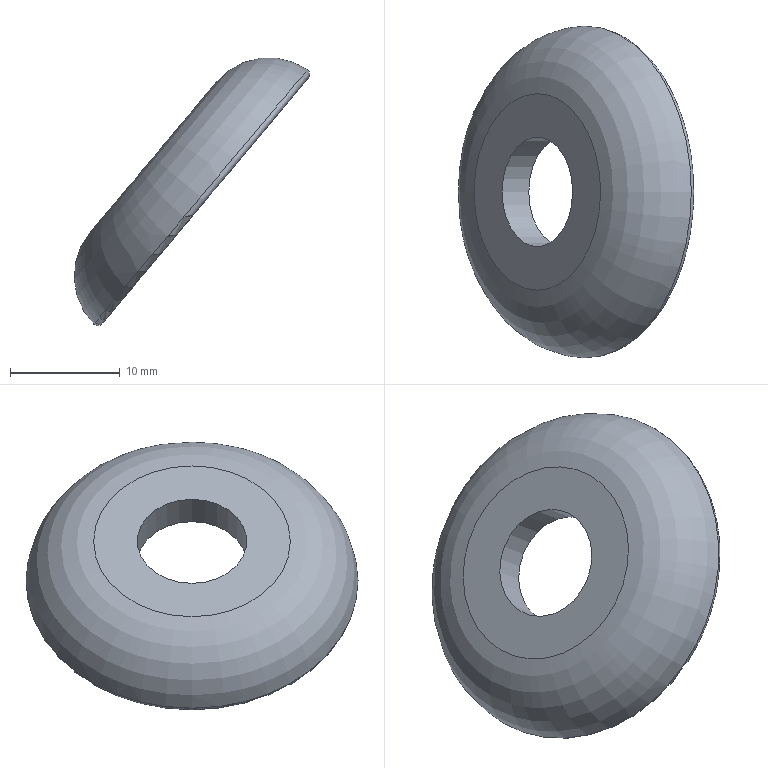Component | NX | BASEWASHER_2 | 1 solid | 9 faces | box 21.48 x 30.3 x 24.46 mm | volume 2198 mm3 | torus 4 | plane 3 | cylinder 2 | commonest cylinder face diameters 10 x1 24 x1
STEP:
#1=CARTESIAN_POINT('',(0.,0.,0.));
#2=DIRECTION('',(0.,0.,1.));
#3=DIRECTION('',(1.,0.,0.));
#4=AXIS2_PLACEMENT_3D('',#1,#2,#3);
#5=CARTESIAN_POINT('',(413.514,0.,-45.75));
#6=VERTEX_POINT('',#5);
#7=CARTESIAN_POINT('',(419.941,0.,-38.089));
#8=DIRECTION('',(0.766,0.,-0.6428));
#9=DIRECTION('',(-0.6428,0.,-0.766));
#10=AXIS2_PLACEMENT_3D('',#7,#8,#9);
#11=CIRCLE('',#10,10.);
#12=CARTESIAN_POINT('',(419.941,0.,-38.089));
#13=DIRECTION('',(0.766,0.,-0.6428));
#14=DIRECTION('',(-0.6428,0.,-0.766));
#15=AXIS2_PLACEMENT_3D('',#12,#13,#14);
#16=PLANE('',#15);
#17=CARTESIAN_POINT('',(-0.,0.));
#18=DIRECTION('',(1.,0.));
#19=AXIS2_PLACEMENT_2D('',#17,#18);
#20=CIRCLE('',#19,10.);
#21=(GEOMETRIC_REPRESENTATION_CONTEXT(2)PARAMETRIC_REPRESENTATION_CONTEXT()REPRESENTATION_CONTEXT('',''));
#22=DEFINITIONAL_REPRESENTATION('',(#20),#21);
#23=PCURVE('',#16,#22);
#24=CARTESIAN_POINT('',(421.473,0.,-39.375));
#25=DIRECTION('',(0.766,0.,-0.6428));
#26=DIRECTION('',(-0.6428,0.,-0.766));
#27=AXIS2_PLACEMENT_3D('',#24,#25,#26);
#28=TOROIDAL_SURFACE('',#27,10.,2.);
#29=CARTESIAN_POINT('',(0.,4.712));
#30=DIRECTION('',(1.,0.));
#31=VECTOR('',#30,1.);
#32=LINE('',#29,#31);
#33=(GEOMETRIC_REPRESENTATION_CONTEXT(2)PARAMETRIC_REPRESENTATION_CONTEXT()REPRESENTATION_CONTEXT('',''));
#34=DEFINITIONAL_REPRESENTATION('',(#32),#33);
#35=PCURVE('',#28,#34);
#36=SURFACE_CURVE('',#11,(#23,#35),.PCURVE_S1.);
#37=EDGE_CURVE('',#6,#6,#36,.T.);
#38=ORIENTED_EDGE('',*,*,#37,.T.);
#39=EDGE_LOOP('',(#38));
#40=FACE_BOUND('',#39,.T.);
#41=CARTESIAN_POINT('',(423.155,0.,-34.259));
#42=VERTEX_POINT('',#41);
#43=CARTESIAN_POINT('',(419.941,0.,-38.089));
#44=DIRECTION('',(-0.766,0.,0.6428));
#45=DIRECTION('',(0.6428,0.,0.766));
#46=AXIS2_PLACEMENT_3D('',#43,#44,#45);
#47=CIRCLE('',#46,5.);
#48=CARTESIAN_POINT('',(-5.,0.));
#49=CARTESIAN_POINT('',(-5.,8.66));
#50=CARTESIAN_POINT('',(2.5,4.33));
#51=CARTESIAN_POINT('',(10.,0.));
#52=CARTESIAN_POINT('',(2.5,-4.33));
#53=CARTESIAN_POINT('',(-5.,-8.66));
#54=CARTESIAN_POINT('',(-5.,0.));
#55=(BOUNDED_CURVE()B_SPLINE_CURVE(2,(#48,#49,#50,#51,#52,#53,#54),.UNSPECIFIED.,.T.,.F.)B_SPLINE_CURVE_WITH_KNOTS((1,2,2,2,2,1),(-2.094,0.,2.094,4.189,6.283,8.378),.UNSPECIFIED.)CURVE()GEOMETRIC_REPRESENTATION_ITEM()RATIONAL_B_SPLINE_CURVE((1.,0.5,1.,0.5,1.,0.5,1.))REPRESENTATION_ITEM(''));
#56=(GEOMETRIC_REPRESENTATION_CONTEXT(2)PARAMETRIC_REPRESENTATION_CONTEXT()REPRESENTATION_CONTEXT('',''));
#57=DEFINITIONAL_REPRESENTATION('',(#55),#56);
#58=PCURVE('',#16,#57);
#59=CARTESIAN_POINT('',(419.941,0.,-38.089));
#60=DIRECTION('',(-0.766,0.,0.6428));
#61=DIRECTION('',(0.6428,0.,0.766));
#62=AXIS2_PLACEMENT_3D('',#59,#60,#61);
#63=CYLINDRICAL_SURFACE('',#62,5.);
#64=CARTESIAN_POINT('',(0.,0.));
#65=DIRECTION('',(1.,0.));
#66=VECTOR('',#65,1.);
#67=LINE('',#64,#66);
#68=(GEOMETRIC_REPRESENTATION_CONTEXT(2)PARAMETRIC_REPRESENTATION_CONTEXT()REPRESENTATION_CONTEXT('',''));
#69=DEFINITIONAL_REPRESENTATION('',(#67),#68);
#70=PCURVE('',#63,#69);
#71=SURFACE_CURVE('',#47,(#58,#70),.PCURVE_S1.);
#72=EDGE_CURVE('',#42,#42,#71,.T.);
#73=ORIENTED_EDGE('',*,*,#72,.T.);
#74=EDGE_LOOP('',(#73));
#75=FACE_BOUND('',#74,.T.);
#76=ADVANCED_FACE('',(#40,#75),#16,.T.);
#77=CARTESIAN_POINT('',(423.278,0.,-29.173));
#78=VERTEX_POINT('',#77);
#79=CARTESIAN_POINT('',(411.74,0.,-42.924));
#80=VERTEX_POINT('',#79);
#81=CARTESIAN_POINT('',(417.509,0.,-36.049));
#82=DIRECTION('',(-0.766,0.,0.6428));
#83=DIRECTION('',(0.6428,0.,0.766));
#84=AXIS2_PLACEMENT_3D('',#81,#82,#83);
#85=CIRCLE('',#84,8.975);
#86=CARTESIAN_POINT('',(417.509,0.,-36.049));
#87=DIRECTION('',(-0.766,0.,0.6428));
#88=DIRECTION('',(0.6428,0.,0.766));
#89=AXIS2_PLACEMENT_3D('',#86,#87,#88);
#90=PLANE('',#89);
#91=CARTESIAN_POINT('',(0.,0.));
#92=DIRECTION('',(1.,0.));
#93=AXIS2_PLACEMENT_2D('',#91,#92);
#94=CIRCLE('',#93,8.975);
#95=(GEOMETRIC_REPRESENTATION_CONTEXT(2)PARAMETRIC_REPRESENTATION_CONTEXT()REPRESENTATION_CONTEXT('',''));
#96=DEFINITIONAL_REPRESENTATION('',(#94),#95);
#97=PCURVE('',#90,#96);
#98=CARTESIAN_POINT('',(422.259,0.,-40.034));
#99=DIRECTION('',(0.766,0.,-0.6428));
#100=DIRECTION('',(-0.6428,0.,-0.766));
#101=AXIS2_PLACEMENT_3D('',#98,#99,#100);
#102=TOROIDAL_SURFACE('',#101,8.975,6.2);
#103=CARTESIAN_POINT('',(3.142,4.712));
#104=DIRECTION('',(-1.,0.));
#105=VECTOR('',#104,1.);
#106=LINE('',#103,#105);
#107=(GEOMETRIC_REPRESENTATION_CONTEXT(2)PARAMETRIC_REPRESENTATION_CONTEXT()REPRESENTATION_CONTEXT('',''));
#108=DEFINITIONAL_REPRESENTATION('',(#106),#107);
#109=PCURVE('',#102,#108);
#110=SURFACE_CURVE('',#85,(#97,#109),.PCURVE_S1.);
#111=EDGE_CURVE('',#78,#80,#110,.T.);
#112=ORIENTED_EDGE('',*,*,#111,.T.);
#113=CARTESIAN_POINT('',(417.509,0.,-36.049));
#114=DIRECTION('',(-0.766,0.,0.6428));
#115=DIRECTION('',(0.6428,0.,0.766));
#116=AXIS2_PLACEMENT_3D('',#113,#114,#115);
#117=CIRCLE('',#116,8.975);
#118=CARTESIAN_POINT('',(0.,0.));
#119=DIRECTION('',(1.,0.));
#120=AXIS2_PLACEMENT_2D('',#118,#119);
#121=CIRCLE('',#120,8.975);
#122=(GEOMETRIC_REPRESENTATION_CONTEXT(2)PARAMETRIC_REPRESENTATION_CONTEXT()REPRESENTATION_CONTEXT('',''));
#123=DEFINITIONAL_REPRESENTATION('',(#121),#122);
#124=PCURVE('',#90,#123);
#125=CARTESIAN_POINT('',(9.425,4.712));
#126=DIRECTION('',(-1.,0.));
#127=VECTOR('',#126,1.);
#128=LINE('',#125,#127);
#129=(GEOMETRIC_REPRESENTATION_CONTEXT(2)PARAMETRIC_REPRESENTATION_CONTEXT()REPRESENTATION_CONTEXT('',''));
#130=DEFINITIONAL_REPRESENTATION('',(#128),#129);
#131=PCURVE('',#102,#130);
#132=SURFACE_CURVE('',#117,(#124,#131),.PCURVE_S1.);
#133=EDGE_CURVE('',#80,#78,#132,.T.);
#134=ORIENTED_EDGE('',*,*,#133,.T.);
#135=EDGE_LOOP('',(#112,#134));
#136=FACE_BOUND('',#135,.T.);
#137=CARTESIAN_POINT('',(420.723,0.,-32.218));
#138=VERTEX_POINT('',#137);
#139=CARTESIAN_POINT('',(417.509,0.,-36.049));
#140=DIRECTION('',(0.766,0.,-0.6428));
#141=DIRECTION('',(0.6428,0.,0.766));
#142=AXIS2_PLACEMENT_3D('',#139,#140,#141);
#143=CIRCLE('',#142,5.);
#144=CARTESIAN_POINT('',(5.,0.));
#145=CARTESIAN_POINT('',(5.,-8.66));
#146=CARTESIAN_POINT('',(-2.5,-4.33));
#147=CARTESIAN_POINT('',(-10.,-0.));
#148=CARTESIAN_POINT('',(-2.5,4.33));
#149=CARTESIAN_POINT('',(5.,8.66));
#150=CARTESIAN_POINT('',(5.,0.));
#151=(BOUNDED_CURVE()B_SPLINE_CURVE(2,(#144,#145,#146,#147,#148,#149,#150),.UNSPECIFIED.,.T.,.F.)B_SPLINE_CURVE_WITH_KNOTS((1,2,2,2,2,1),(-2.094,0.,2.094,4.189,6.283,8.378),.UNSPECIFIED.)CURVE()GEOMETRIC_REPRESENTATION_ITEM()RATIONAL_B_SPLINE_CURVE((1.,0.5,1.,0.5,1.,0.5,1.))REPRESENTATION_ITEM(''));
#152=(GEOMETRIC_REPRESENTATION_CONTEXT(2)PARAMETRIC_REPRESENTATION_CONTEXT()REPRESENTATION_CONTEXT('',''));
#153=DEFINITIONAL_REPRESENTATION('',(#151),#152);
#154=PCURVE('',#90,#153);
#155=CARTESIAN_POINT('',(6.283,3.175));
#156=DIRECTION('',(-1.,0.));
#157=VECTOR('',#156,1.);
#158=LINE('',#155,#157);
#159=(GEOMETRIC_REPRESENTATION_CONTEXT(2)PARAMETRIC_REPRESENTATION_CONTEXT()REPRESENTATION_CONTEXT('',''));
#160=DEFINITIONAL_REPRESENTATION('',(#158),#159);
#161=PCURVE('',#63,#160);
#162=SURFACE_CURVE('',#143,(#154,#161),.PCURVE_S1.);
#163=EDGE_CURVE('',#138,#138,#162,.T.);
#164=ORIENTED_EDGE('',*,*,#163,.T.);
#165=EDGE_LOOP('',(#164));
#166=FACE_BOUND('',#165,.T.);
#167=ADVANCED_FACE('',(#136,#166),#90,.T.);
#168=ORIENTED_EDGE('',*,*,#163,.T.);
#169=CARTESIAN_POINT('',(423.155,-0.,-34.259));
#170=CARTESIAN_POINT('',(420.723,-0.,-32.218));
#171=B_SPLINE_CURVE_WITH_KNOTS('',1,(#169,#170),.UNSPECIFIED.,.F.,.F.,(2,2),(0.,3.175),.PIECEWISE_BEZIER_KNOTS.);
#172=CARTESIAN_POINT('',(0.,0.));
#173=DIRECTION('',(0.,1.));
#174=VECTOR('',#173,1.);
#175=LINE('',#172,#174);
#176=(GEOMETRIC_REPRESENTATION_CONTEXT(2)PARAMETRIC_REPRESENTATION_CONTEXT()REPRESENTATION_CONTEXT('',''));
#177=DEFINITIONAL_REPRESENTATION('',(#175),#176);
#178=PCURVE('',#63,#177);
#179=CARTESIAN_POINT('',(6.283,0.));
#180=DIRECTION('',(0.,1.));
#181=VECTOR('',#180,1.);
#182=LINE('',#179,#181);
#183=(GEOMETRIC_REPRESENTATION_CONTEXT(2)PARAMETRIC_REPRESENTATION_CONTEXT()REPRESENTATION_CONTEXT('',''));
#184=DEFINITIONAL_REPRESENTATION('',(#182),#183);
#185=PCURVE('',#63,#184);
#186=SEAM_CURVE('',#171,(#178,#185),.PCURVE_S1.);
#187=EDGE_CURVE('',#42,#138,#186,.T.);
#188=ORIENTED_EDGE('',*,*,#187,.F.);
#189=ORIENTED_EDGE('',*,*,#72,.T.);
#190=ORIENTED_EDGE('',*,*,#187,.T.);
#191=EDGE_LOOP('',(#168,#188,#189,#190));
#192=FACE_BOUND('',#191,.F.);
#193=ADVANCED_FACE('',(#192),#63,.F.);
#194=CARTESIAN_POINT('',(414.143,0.,-48.889));
#195=VERTEX_POINT('',#194);
#196=CARTESIAN_POINT('',(421.857,0.,-39.696));
#197=DIRECTION('',(0.766,0.,-0.6428));
#198=DIRECTION('',(-0.6428,0.,-0.766));
#199=AXIS2_PLACEMENT_3D('',#196,#197,#198);
#200=CIRCLE('',#199,12.);
#201=CARTESIAN_POINT('',(419.941,0.,-38.089));
#202=DIRECTION('',(0.766,0.,-0.6428));
#203=DIRECTION('',(-0.6428,0.,-0.766));
#204=AXIS2_PLACEMENT_3D('',#201,#202,#203);
#205=CYLINDRICAL_SURFACE('',#204,12.);
#206=CARTESIAN_POINT('',(0.,2.5));
#207=DIRECTION('',(1.,0.));
#208=VECTOR('',#207,1.);
#209=LINE('',#206,#208);
#210=(GEOMETRIC_REPRESENTATION_CONTEXT(2)PARAMETRIC_REPRESENTATION_CONTEXT()REPRESENTATION_CONTEXT('',''));
#211=DEFINITIONAL_REPRESENTATION('',(#209),#210);
#212=PCURVE('',#205,#211);
#213=CARTESIAN_POINT('',(421.857,0.,-39.696));
#214=DIRECTION('',(0.766,0.,-0.6428));
#215=DIRECTION('',(-0.6428,0.,-0.766));
#216=AXIS2_PLACEMENT_3D('',#213,#214,#215);
#217=TOROIDAL_SURFACE('',#216,12.5,0.5);
#218=CARTESIAN_POINT('',(0.,9.425));
#219=DIRECTION('',(1.,0.));
#220=VECTOR('',#219,1.);
#221=LINE('',#218,#220);
#222=(GEOMETRIC_REPRESENTATION_CONTEXT(2)PARAMETRIC_REPRESENTATION_CONTEXT()REPRESENTATION_CONTEXT('',''));
#223=DEFINITIONAL_REPRESENTATION('',(#221),#222);
#224=PCURVE('',#217,#223);
#225=SURFACE_CURVE('',#200,(#212,#224),.PCURVE_S1.);
#226=EDGE_CURVE('',#195,#195,#225,.T.);
#227=ORIENTED_EDGE('',*,*,#226,.F.);
#228=CARTESIAN_POINT('',(413.76,0.,-48.568));
#229=VERTEX_POINT('',#228);
#230=CARTESIAN_POINT('',(413.76,-0.,-48.568));
#231=CARTESIAN_POINT('',(414.143,-0.,-48.889));
#232=B_SPLINE_CURVE_WITH_KNOTS('',1,(#230,#231),.UNSPECIFIED.,.F.,.F.,(2,2),(2.,2.5),.PIECEWISE_BEZIER_KNOTS.);
#233=CARTESIAN_POINT('',(0.,0.));
#234=DIRECTION('',(0.,1.));
#235=VECTOR('',#234,1.);
#236=LINE('',#233,#235);
#237=(GEOMETRIC_REPRESENTATION_CONTEXT(2)PARAMETRIC_REPRESENTATION_CONTEXT()REPRESENTATION_CONTEXT('',''));
#238=DEFINITIONAL_REPRESENTATION('',(#236),#237);
#239=PCURVE('',#205,#238);
#240=CARTESIAN_POINT('',(6.283,0.));
#241=DIRECTION('',(0.,1.));
#242=VECTOR('',#241,1.);
#243=LINE('',#240,#242);
#244=(GEOMETRIC_REPRESENTATION_CONTEXT(2)PARAMETRIC_REPRESENTATION_CONTEXT()REPRESENTATION_CONTEXT('',''));
#245=DEFINITIONAL_REPRESENTATION('',(#243),#244);
#246=PCURVE('',#205,#245);
#247=SEAM_CURVE('',#232,(#239,#246),.PCURVE_S1.);
#248=EDGE_CURVE('',#229,#195,#247,.T.);
#249=ORIENTED_EDGE('',*,*,#248,.F.);
#250=CARTESIAN_POINT('',(421.473,0.,-39.375));
#251=DIRECTION('',(-0.766,0.,0.6428));
#252=DIRECTION('',(-0.6428,0.,-0.766));
#253=AXIS2_PLACEMENT_3D('',#250,#251,#252);
#254=CIRCLE('',#253,12.);
#255=CARTESIAN_POINT('',(6.283,2.));
#256=DIRECTION('',(-1.,0.));
#257=VECTOR('',#256,1.);
#258=LINE('',#255,#257);
#259=(GEOMETRIC_REPRESENTATION_CONTEXT(2)PARAMETRIC_REPRESENTATION_CONTEXT()REPRESENTATION_CONTEXT('',''));
#260=DEFINITIONAL_REPRESENTATION('',(#258),#259);
#261=PCURVE('',#205,#260);
#262=CARTESIAN_POINT('',(6.283,6.283));
#263=DIRECTION('',(-1.,0.));
#264=VECTOR('',#263,1.);
#265=LINE('',#262,#264);
#266=(GEOMETRIC_REPRESENTATION_CONTEXT(2)PARAMETRIC_REPRESENTATION_CONTEXT()REPRESENTATION_CONTEXT('',''));
#267=DEFINITIONAL_REPRESENTATION('',(#265),#266);
#268=PCURVE('',#28,#267);
#269=SURFACE_CURVE('',#254,(#261,#268),.PCURVE_S1.);
#270=EDGE_CURVE('',#229,#229,#269,.T.);
#271=ORIENTED_EDGE('',*,*,#270,.F.);
#272=ORIENTED_EDGE('',*,*,#248,.T.);
#273=EDGE_LOOP('',(#227,#249,#271,#272));
#274=FACE_BOUND('',#273,.F.);
#275=ADVANCED_FACE('',(#274),#205,.F.);
#276=CARTESIAN_POINT('',(414.205,0.,-49.593));
#277=VERTEX_POINT('',#276);
#278=CARTESIAN_POINT('',(422.24,0.,-40.018));
#279=DIRECTION('',(-0.766,0.,0.6428));
#280=DIRECTION('',(-0.6428,0.,-0.766));
#281=AXIS2_PLACEMENT_3D('',#278,#279,#280);
#282=CIRCLE('',#281,12.5);
#283=CARTESIAN_POINT('',(414.526,0.,-49.21));
#284=DIRECTION('',(0.766,0.,-0.6428));
#285=DIRECTION('',(-0.6428,0.,-0.766));
#286=AXIS2_PLACEMENT_3D('',#283,#284,#285);
#287=PLANE('',#286);
#288=CARTESIAN_POINT('',(0.5,0.));
#289=CARTESIAN_POINT('',(0.5,-21.651));
#290=CARTESIAN_POINT('',(-18.25,-10.825));
#291=CARTESIAN_POINT('',(-37.,-0.));
#292=CARTESIAN_POINT('',(-18.25,10.825));
#293=CARTESIAN_POINT('',(0.5,21.651));
#294=CARTESIAN_POINT('',(0.5,0.));
#295=(BOUNDED_CURVE()B_SPLINE_CURVE(2,(#288,#289,#290,#291,#292,#293,#294),.UNSPECIFIED.,.T.,.F.)B_SPLINE_CURVE_WITH_KNOTS((1,2,2,2,2,1),(-2.094,0.,2.094,4.189,6.283,8.378),.UNSPECIFIED.)CURVE()GEOMETRIC_REPRESENTATION_ITEM()RATIONAL_B_SPLINE_CURVE((1.,0.5,1.,0.5,1.,0.5,1.))REPRESENTATION_ITEM(''));
#296=(GEOMETRIC_REPRESENTATION_CONTEXT(2)PARAMETRIC_REPRESENTATION_CONTEXT()REPRESENTATION_CONTEXT('',''));
#297=DEFINITIONAL_REPRESENTATION('',(#295),#296);
#298=PCURVE('',#287,#297);
#299=CARTESIAN_POINT('',(6.283,7.854));
#300=DIRECTION('',(-1.,0.));
#301=VECTOR('',#300,1.);
#302=LINE('',#299,#301);
#303=(GEOMETRIC_REPRESENTATION_CONTEXT(2)PARAMETRIC_REPRESENTATION_CONTEXT()REPRESENTATION_CONTEXT('',''));
#304=DEFINITIONAL_REPRESENTATION('',(#302),#303);
#305=PCURVE('',#217,#304);
#306=SURFACE_CURVE('',#282,(#298,#305),.PCURVE_S1.);
#307=EDGE_CURVE('',#277,#277,#306,.T.);
#308=ORIENTED_EDGE('',*,*,#307,.T.);
#309=EDGE_LOOP('',(#308));
#310=FACE_BOUND('',#309,.T.);
#311=CARTESIAN_POINT('',(412.822,0.,-51.241));
#312=VERTEX_POINT('',#311);
#313=CARTESIAN_POINT('',(422.24,0.,-40.018));
#314=DIRECTION('',(0.766,0.,-0.6428));
#315=DIRECTION('',(-0.6428,0.,-0.766));
#316=AXIS2_PLACEMENT_3D('',#313,#314,#315);
#317=CIRCLE('',#316,14.651);
#318=CARTESIAN_POINT('',(-12.,0.));
#319=DIRECTION('',(1.,0.));
#320=AXIS2_PLACEMENT_2D('',#318,#319);
#321=CIRCLE('',#320,14.651);
#322=(GEOMETRIC_REPRESENTATION_CONTEXT(2)PARAMETRIC_REPRESENTATION_CONTEXT()REPRESENTATION_CONTEXT('',''));
#323=DEFINITIONAL_REPRESENTATION('',(#321),#322);
#324=PCURVE('',#287,#323);
#325=CARTESIAN_POINT('',(421.857,0.,-39.696));
#326=DIRECTION('',(0.766,0.,-0.6428));
#327=DIRECTION('',(-0.6428,0.,-0.766));
#328=AXIS2_PLACEMENT_3D('',#325,#326,#327);
#329=TOROIDAL_SURFACE('',#328,14.651,0.5);
#330=CARTESIAN_POINT('',(0.,7.854));
#331=DIRECTION('',(1.,0.));
#332=VECTOR('',#331,1.);
#333=LINE('',#330,#332);
#334=(GEOMETRIC_REPRESENTATION_CONTEXT(2)PARAMETRIC_REPRESENTATION_CONTEXT()REPRESENTATION_CONTEXT('',''));
#335=DEFINITIONAL_REPRESENTATION('',(#333),#334);
#336=PCURVE('',#329,#335);
#337=SURFACE_CURVE('',#317,(#324,#336),.PCURVE_S1.);
#338=EDGE_CURVE('',#312,#312,#337,.T.);
#339=ORIENTED_EDGE('',*,*,#338,.T.);
#340=EDGE_LOOP('',(#339));
#341=FACE_BOUND('',#340,.T.);
#342=ADVANCED_FACE('',(#310,#341),#287,.T.);
#343=ORIENTED_EDGE('',*,*,#37,.T.);
#344=CARTESIAN_POINT('',(413.514,0.,-45.75));
#345=CARTESIAN_POINT('',(413.17,0.,-46.159));
#346=CARTESIAN_POINT('',(412.965,0.,-46.668));
#347=CARTESIAN_POINT('',(412.927,0.,-47.221));
#348=CARTESIAN_POINT('',(413.061,0.,-47.759));
#349=CARTESIAN_POINT('',(413.35,0.,-48.224));
#350=CARTESIAN_POINT('',(413.76,0.,-48.568));
#351=(BOUNDED_CURVE()B_SPLINE_CURVE(6,(#344,#345,#346,#347,#348,#349,#350),.UNSPECIFIED.,.F.,.F.)B_SPLINE_CURVE_WITH_KNOTS((7,7),(4.712,6.283),.PIECEWISE_BEZIER_KNOTS.)CURVE()GEOMETRIC_REPRESENTATION_ITEM()RATIONAL_B_SPLINE_CURVE((1.031,1.01,0.9979,0.994,0.9979,1.01,1.031))REPRESENTATION_ITEM(''));
#352=CARTESIAN_POINT('',(6.283,0.));
#353=DIRECTION('',(0.,1.));
#354=VECTOR('',#353,1.);
#355=LINE('',#352,#354);
#356=(GEOMETRIC_REPRESENTATION_CONTEXT(2)PARAMETRIC_REPRESENTATION_CONTEXT()REPRESENTATION_CONTEXT('',''));
#357=DEFINITIONAL_REPRESENTATION('',(#355),#356);
#358=PCURVE('',#28,#357);
#359=CARTESIAN_POINT('',(0.,0.));
#360=DIRECTION('',(0.,1.));
#361=VECTOR('',#360,1.);
#362=LINE('',#359,#361);
#363=(GEOMETRIC_REPRESENTATION_CONTEXT(2)PARAMETRIC_REPRESENTATION_CONTEXT()REPRESENTATION_CONTEXT('',''));
#364=DEFINITIONAL_REPRESENTATION('',(#362),#363);
#365=PCURVE('',#28,#364);
#366=SEAM_CURVE('',#351,(#358,#365),.PCURVE_S1.);
#367=EDGE_CURVE('',#6,#229,#366,.T.);
#368=ORIENTED_EDGE('',*,*,#367,.T.);
#369=ORIENTED_EDGE('',*,*,#270,.T.);
#370=ORIENTED_EDGE('',*,*,#367,.F.);
#371=EDGE_LOOP('',(#343,#368,#369,#370));
#372=FACE_BOUND('',#371,.F.);
#373=ADVANCED_FACE('',(#372),#28,.F.);
#374=CARTESIAN_POINT('',(412.084,0.,-51.271));
#375=VERTEX_POINT('',#374);
#376=CARTESIAN_POINT('',(421.821,0.,-39.667));
#377=DIRECTION('',(-0.766,0.,0.6428));
#378=DIRECTION('',(-0.6428,0.,-0.766));
#379=AXIS2_PLACEMENT_3D('',#376,#377,#378);
#380=CIRCLE('',#379,15.149);
#381=CARTESIAN_POINT('',(6.283,6.191));
#382=DIRECTION('',(-1.,0.));
#383=VECTOR('',#382,1.);
#384=LINE('',#381,#383);
#385=(GEOMETRIC_REPRESENTATION_CONTEXT(2)PARAMETRIC_REPRESENTATION_CONTEXT()REPRESENTATION_CONTEXT('',''));
#386=DEFINITIONAL_REPRESENTATION('',(#384),#385);
#387=PCURVE('',#102,#386);
#388=CARTESIAN_POINT('',(6.283,6.191));
#389=DIRECTION('',(-1.,0.));
#390=VECTOR('',#389,1.);
#391=LINE('',#388,#390);
#392=(GEOMETRIC_REPRESENTATION_CONTEXT(2)PARAMETRIC_REPRESENTATION_CONTEXT()REPRESENTATION_CONTEXT('',''));
#393=DEFINITIONAL_REPRESENTATION('',(#391),#392);
#394=PCURVE('',#329,#393);
#395=SURFACE_CURVE('',#380,(#387,#394),.PCURVE_S1.);
#396=EDGE_CURVE('',#375,#375,#395,.T.);
#397=ORIENTED_EDGE('',*,*,#396,.T.);
#398=CARTESIAN_POINT('',(411.74,-0.,-42.924));
#399=CARTESIAN_POINT('',(410.74,-0.,-44.116));
#400=CARTESIAN_POINT('',(410.119,-0.,-45.58));
#401=CARTESIAN_POINT('',(409.948,-0.,-47.179));
#402=CARTESIAN_POINT('',(410.249,-0.,-48.757));
#403=CARTESIAN_POINT('',(410.989,-0.,-50.165));
#404=CARTESIAN_POINT('',(412.084,-0.,-51.271));
#405=(BOUNDED_CURVE()B_SPLINE_CURVE(6,(#398,#399,#400,#401,#402,#403,#404),.UNSPECIFIED.,.F.,.F.)B_SPLINE_CURVE_WITH_KNOTS((7,7),(4.712,6.191),.PIECEWISE_BEZIER_KNOTS.)CURVE()GEOMETRIC_REPRESENTATION_ITEM()RATIONAL_B_SPLINE_CURVE((1.028,1.009,0.9982,0.9946,0.9982,1.009,1.028))REPRESENTATION_ITEM(''));
#406=CARTESIAN_POINT('',(0.,0.));
#407=DIRECTION('',(0.,1.));
#408=VECTOR('',#407,1.);
#409=LINE('',#406,#408);
#410=(GEOMETRIC_REPRESENTATION_CONTEXT(2)PARAMETRIC_REPRESENTATION_CONTEXT()REPRESENTATION_CONTEXT('',''));
#411=DEFINITIONAL_REPRESENTATION('',(#409),#410);
#412=PCURVE('',#102,#411);
#413=CARTESIAN_POINT('',(6.283,0.));
#414=DIRECTION('',(0.,1.));
#415=VECTOR('',#414,1.);
#416=LINE('',#413,#415);
#417=(GEOMETRIC_REPRESENTATION_CONTEXT(2)PARAMETRIC_REPRESENTATION_CONTEXT()REPRESENTATION_CONTEXT('',''));
#418=DEFINITIONAL_REPRESENTATION('',(#416),#417);
#419=PCURVE('',#102,#418);
#420=SEAM_CURVE('',#405,(#412,#419),.PCURVE_S1.);
#421=EDGE_CURVE('',#80,#375,#420,.T.);
#422=ORIENTED_EDGE('',*,*,#421,.F.);
#423=ORIENTED_EDGE('',*,*,#111,.F.);
#424=ORIENTED_EDGE('',*,*,#133,.F.);
#425=ORIENTED_EDGE('',*,*,#421,.T.);
#426=EDGE_LOOP('',(#397,#422,#423,#424,#425));
#427=FACE_BOUND('',#426,.T.);
#428=ADVANCED_FACE('',(#427),#102,.T.);
#429=ORIENTED_EDGE('',*,*,#307,.F.);
#430=CARTESIAN_POINT('',(414.205,0.,-49.593));
#431=CARTESIAN_POINT('',(414.291,0.,-49.491));
#432=CARTESIAN_POINT('',(414.342,0.,-49.364));
#433=CARTESIAN_POINT('',(414.351,0.,-49.226));
#434=CARTESIAN_POINT('',(414.318,0.,-49.091));
#435=CARTESIAN_POINT('',(414.245,0.,-48.975));
#436=CARTESIAN_POINT('',(414.143,0.,-48.889));
#437=(BOUNDED_CURVE()B_SPLINE_CURVE(6,(#430,#431,#432,#433,#434,#435,#436),.UNSPECIFIED.,.F.,.F.)B_SPLINE_CURVE_WITH_KNOTS((7,7),(1.571,3.142),.PIECEWISE_BEZIER_KNOTS.)CURVE()GEOMETRIC_REPRESENTATION_ITEM()RATIONAL_B_SPLINE_CURVE((1.031,1.01,0.9979,0.994,0.9979,1.01,1.031))REPRESENTATION_ITEM(''));
#438=CARTESIAN_POINT('',(6.283,6.283));
#439=DIRECTION('',(0.,1.));
#440=VECTOR('',#439,1.);
#441=LINE('',#438,#440);
#442=(GEOMETRIC_REPRESENTATION_CONTEXT(2)PARAMETRIC_REPRESENTATION_CONTEXT()REPRESENTATION_CONTEXT('',''));
#443=DEFINITIONAL_REPRESENTATION('',(#441),#442);
#444=PCURVE('',#217,#443);
#445=CARTESIAN_POINT('',(0.,6.283));
#446=DIRECTION('',(0.,1.));
#447=VECTOR('',#446,1.);
#448=LINE('',#445,#447);
#449=(GEOMETRIC_REPRESENTATION_CONTEXT(2)PARAMETRIC_REPRESENTATION_CONTEXT()REPRESENTATION_CONTEXT('',''));
#450=DEFINITIONAL_REPRESENTATION('',(#448),#449);
#451=PCURVE('',#217,#450);
#452=SEAM_CURVE('',#437,(#444,#451),.PCURVE_S1.);
#453=EDGE_CURVE('',#277,#195,#452,.T.);
#454=ORIENTED_EDGE('',*,*,#453,.T.);
#455=ORIENTED_EDGE('',*,*,#226,.F.);
#456=ORIENTED_EDGE('',*,*,#453,.F.);
#457=EDGE_LOOP('',(#429,#454,#455,#456));
#458=FACE_BOUND('',#457,.T.);
#459=ADVANCED_FACE('',(#458),#217,.T.);
#460=ORIENTED_EDGE('',*,*,#396,.F.);
#461=CARTESIAN_POINT('',(412.084,0.,-51.271));
#462=CARTESIAN_POINT('',(412.181,0.,-51.37));
#463=CARTESIAN_POINT('',(412.312,0.,-51.436));
#464=CARTESIAN_POINT('',(412.461,0.,-51.456));
#465=CARTESIAN_POINT('',(412.609,0.,-51.424));
#466=CARTESIAN_POINT('',(412.733,0.,-51.347));
#467=CARTESIAN_POINT('',(412.822,0.,-51.241));
#468=B_SPLINE_CURVE_WITH_KNOTS('',6,(#461,#462,#463,#464,#465,#466,#467),.UNSPECIFIED.,.F.,.F.,(7,7),(6.191,7.854),.PIECEWISE_BEZIER_KNOTS.);
#469=CARTESIAN_POINT('',(6.283,0.));
#470=DIRECTION('',(0.,1.));
#471=VECTOR('',#470,1.);
#472=LINE('',#469,#471);
#473=(GEOMETRIC_REPRESENTATION_CONTEXT(2)PARAMETRIC_REPRESENTATION_CONTEXT()REPRESENTATION_CONTEXT('',''));
#474=DEFINITIONAL_REPRESENTATION('',(#472),#473);
#475=PCURVE('',#329,#474);
#476=CARTESIAN_POINT('',(0.,0.));
#477=DIRECTION('',(0.,1.));
#478=VECTOR('',#477,1.);
#479=LINE('',#476,#478);
#480=(GEOMETRIC_REPRESENTATION_CONTEXT(2)PARAMETRIC_REPRESENTATION_CONTEXT()REPRESENTATION_CONTEXT('',''));
#481=DEFINITIONAL_REPRESENTATION('',(#479),#480);
#482=PCURVE('',#329,#481);
#483=SEAM_CURVE('',#468,(#475,#482),.PCURVE_S1.);
#484=EDGE_CURVE('',#375,#312,#483,.T.);
#485=ORIENTED_EDGE('',*,*,#484,.T.);
#486=ORIENTED_EDGE('',*,*,#338,.F.);
#487=ORIENTED_EDGE('',*,*,#484,.F.);
#488=EDGE_LOOP('',(#460,#485,#486,#487));
#489=FACE_BOUND('',#488,.T.);
#490=ADVANCED_FACE('',(#489),#329,.T.);
#491=CLOSED_SHELL('',(#76,#167,#193,#275,#342,#373,#428,#459,#490));
#492=MANIFOLD_SOLID_BREP('',#491);
#493=(LENGTH_UNIT()NAMED_UNIT(*)SI_UNIT(.MILLI.,.METRE.));
#494=UNCERTAINTY_MEASURE_WITH_UNIT(LENGTH_MEASURE(0.00001),#493,'','');
#495=(NAMED_UNIT(*)PLANE_ANGLE_UNIT()SI_UNIT($,.RADIAN.));
#496=(NAMED_UNIT(*)SI_UNIT($,.STERADIAN.)SOLID_ANGLE_UNIT());
#497=(GEOMETRIC_REPRESENTATION_CONTEXT(3)GLOBAL_UNCERTAINTY_ASSIGNED_CONTEXT((#494))GLOBAL_UNIT_ASSIGNED_CONTEXT((#493,#495,#496))REPRESENTATION_CONTEXT('',''));
#498=ADVANCED_BREP_SHAPE_REPRESENTATION('',(#4,#492),#497);